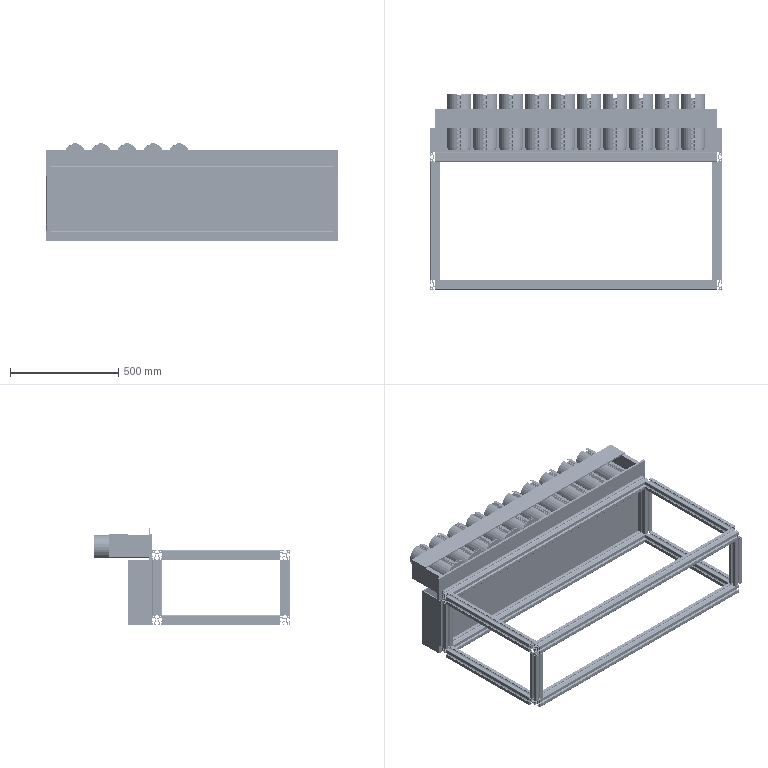Assembly | SolidWorks | mm | 438 component files | 477 solids | 23460 faces | box 1345 x 901.5 x 452.95 mm | volume 26250430 mm3 | cylinder 12408 | plane 6340 | torus 3280 | spline 860 | cone 572 | commonest cylinder face diameters 1 x1650 2.5 x1640 2 x1246 95.6 x1230 98.4 x1230 10 x976 6 x844 3.2 x820
Bill of materials:
Cover | 1 |  | Long, narrow, thin-walled rectangular trough or tray. A tall long wall runs the full length, with a closed end wall at each end and a bottom panel. The top and the long front side look open.
FeedingMechanism | 1 |  | Multi-body geometry: an open rectangular box frame made of slotted profile bars, with a long rectangular housing along one top edge that holds a row of evenly spaced parallel cylinders. A flat panel runs along one long side of the frame under the housing.
PusherTray | 2 |  | Long angle profile with an L-shaped cross-section: a tall thin vertical leg and a short horizontal foot, joined by a rounded inside and outside corner. The top of the tall leg narrows over a short taper.
5 | 4 |  | Socket-head-style fastener shape: a cylindrical head with a hexagonal recess and chamfered edges, on top of a shorter, smaller-diameter plain cylindrical shank with a chamfered tip.
6 | 4 |  | Elongated rectangular-section bar with rounded edges and a smaller cylindrical stub at one end. A thin strip and a small pin- or nut-like feature run along one side. The end view shows a rounded rectangular outline with a narrower raised tab carrying a chamfered cylindrical boss with a slot.
TR-20x75-SBaffle | 4 |  | Solid rectangular block with four through-holes on one face, in a row: a small hole near each end and two larger holes further in. One of the larger holes looks stepped (counterbored or shouldered).
TR-20x75-SCylinderBody | 4 |  | Rectangular body with lengthwise grooves on its long faces and two T-shaped undercut slots in one end profile. Two counterbored round openings and a hex-shaped fitting stick out of the top end. Small holes are spread over the side faces.
TR-20x75-SCylinderRod | 4 |  | Long, slender, solid cylindrical pin with a wider grooved collar at one end and a small notch or flat near the opposite tip. Seen end-on, the collar is circular, with a central section showing two parallel flats.
TR-20x75-SGuideRod | 4 |  | Long, slender tube-like pin, similar in shape to a grooved-collar pin. It has a central bore visible at the tip and a cone-bottomed bore seen from the end. The collar section shows a hexagon-like faceted outline.
WuliangyeBottleCap-1 | 410 |  | Thin flat plate with a mostly circular outline, a small rounded lobe at the top joined by concave fillets, and a straight-sided rectangular tab at the bottom. There are small holes near the tab corners.
Mates:
1. width | PusherTray-1 face at (575, 622.5, 22.5) dir (1, 0, 0) | PusherTray-1 face at (25, 628.5, 22.5) dir (-1, 0, 0) | FeedingMechanism-1 face at (452, 627.5, -157.5) dir (1, 0, 0) | FeedingMechanism-1 face at (148, 627.5, -157.5) dir (-1, 0, 0)
2. width | PusherTray-2 face at (-575, 628.5, 66.449) dir (-1, 0, 0) | PusherTray-2 face at (-25, 622.5, 66.449) dir (1, 0, 0) | FeedingMechanism-1 face at (-452, 627.5, -157.5) dir (-1, 0, 0) | FeedingMechanism-1 face at (-148, 627.5, -157.5) dir (1, 0, 0)
3. coincident | FeedingMechanism-1 face at (0, 622.5, 0) dir (0, 1, 0) | WuliangyeBottleCap-1-1 face at (517.1, 622.5, 143.39) dir (0, -1, 0)
4. concentric | FeedingMechanism-1 face at (540, 879, 187.5) dir (0, -1, 0) r 50 | WuliangyeBottleCap-1-1 face at (540, 622.5, 187.5) dir (0, 1, 0) r 49.2
5. parallel | FeedingMechanism-1 face at (0, 0, 247.479) dir (0, 0, 1) | WuliangyeBottleCap-1-387 face at (517.6, 856.5, 136.695) dir (0, 0, -1)
6. coincident | FeedingMechanism-1 face at (0, 627.5, 0) dir (0, 1, 0) | TR-20x75-S-GN-1 (0)1-1/TR-20x75-SCylinderBody-1 face at (-187.5, 627.5, -7.5) dir (0, -1, 0)
7. coincident | FeedingMechanism-1 edge at (-148, 622.5, -157.5) dir (-1, 0, 0) | TR-20x75-S-GN-1 (0)1-1/TR-20x75-SCylinderBody-1 face at (-180, 627.5, -157.5) dir (0, 0, -1)
8. coincident | FeedingMechanism-1 face at (-148, 627.5, -157.5) dir (1, 0, 0) | TR-20x75-S-GN-1 (0)1-1/TR-20x75-SCylinderBody-1 face at (-148, 628.2, -7.5) dir (1, 0, 0)
9. coincident | PusherTray-2 face at (-575, 628, 60.449) dir (0, 0, -1) | TR-20x75-S-GN-1 (0)1-1/TR-20x75-SBaffle-1 face at (-180, 628.5, 60.449) dir (0, 0, 1)
10. coincident | FeedingMechanism-1 face at (0, 627.5, 0) dir (0, 1, 0) | TR-20x75-S-GN-1 (0)1-2/TR-20x75-SCylinderBody-1 face at (-427.5, 627.5, -7.5) dir (0, -1, 0)
11. coincident | FeedingMechanism-1 face at (-388, 627.5, -157.5) dir (1, 0, 0) | TR-20x75-S-GN-1 (0)1-2/TR-20x75-SCylinderBody-1 face at (-388, 628.2, -7.5) dir (1, 0, 0)
12. coincident | FeedingMechanism-1 face at (-452, 627.5, -7.5) dir (0, 0, 1) | TR-20x75-S-GN-1 (0)1-2/TR-20x75-SCylinderBody-1 face at (-420, 627.5, -7.5) dir (0, 0, 1)
13. coincident | PusherTray-2 face at (-575, 651.5, 60.449) dir (0, 1, 0) | TR-20x75-S-GN-1 (0)1-2/TR-20x75-SBaffle-1 face at (-389.2, 651.5, 60.449) dir (0, 1, 0)
14. coincident | FeedingMechanism-1 face at (0, 627.5, 0) dir (0, 1, 0) | TR-20x75-S-GN-1 (0)-3/TR-20x75-SCylinderBody-1 face at (172.5, 627.5, -7.5) dir (0, -1, 0)
15. coincident | FeedingMechanism-1 face at (212, 627.5, -7.5) dir (0, 0, 1) | TR-20x75-S-GN-1 (0)-3/TR-20x75-SCylinderBody-1 face at (180, 627.5, -7.5) dir (0, 0, 1)
16. coincident | FeedingMechanism-1 face at (212, 627.5, -157.5) dir (1, 0, 0) | TR-20x75-S-GN-1 (0)-3/TR-20x75-SCylinderBody-1 face at (212, 628.2, -7.5) dir (1, 0, 0)
17. coincident | FeedingMechanism-1 face at (0, 627.5, 0) dir (0, 1, 0) | TR-20x75-S-GN-1 (0)-4/TR-20x75-SCylinderBody-1 face at (412.5, 627.5, -7.5) dir (0, -1, 0)
18. coincident | FeedingMechanism-1 face at (452, 627.5, -157.5) dir (1, 0, 0) | TR-20x75-S-GN-1 (0)-4/TR-20x75-SCylinderBody-1 face at (452, 628.2, -7.5) dir (1, 0, 0)
19. coincident | FeedingMechanism-1 face at (452, 627.5, -7.5) dir (0, 0, 1) | TR-20x75-S-GN-1 (0)-4/TR-20x75-SCylinderBody-1 face at (420, 627.5, -7.5) dir (0, 0, 1)
20. coincident | PusherTray-1 face at (25, 628, 16.5) dir (0, 0, -1) | TR-20x75-S-GN-1 (0)-4/TR-20x75-SBaffle-1 face at (420, 628.5, 16.5) dir (0, 0, 1)
21. coincident | PusherTray-1 face at (25, 651.5, 16.5) dir (0, 1, 0) | TR-20x75-S-GN-1 (0)-4/TR-20x75-SBaffle-1 face at (450.8, 651.5, 16.5) dir (0, 1, 0)
22. distance | WuliangyeBottleCap-1-401 face at (-82.9, 628.5, 143.39) dir (0, -1, 0) | FeedingMechanism-1 face at (0, 622.5, 0) dir (0, 1, 0)
23. concentric | FeedingMechanism-1 face at (-60, 879, 187.5) dir (0, -1, 0) r 50 | WuliangyeBottleCap-1-401 face at (-60, 628.5, 187.5) dir (0, 1, 0) r 49.2
24. parallel | FeedingMechanism-1 face at (-672.5, 622.5, 247.5) dir (0, 0, 1) | WuliangyeBottleCap-1-401 face at (-82.4, 628.5, 136.695) dir (0, 0, -1)
25. coincident | FeedingMechanism-1 face at (0, 622.5, 0) dir (0, 1, 0) | WuliangyeBottleCap-1-649 face at (-82.886, 622.5, 182.644) dir (0, -1, 0)
26. coincident | PusherTray-2 face at (-575, 628, 175.949) dir (0, 0, 1) | WuliangyeBottleCap-1-649 face at (-82.386, 622.5, 175.949) dir (0, 0, -1)
27. coincident | FeedingMechanism-1 face at (0, 622.5, 0) dir (0, 1, 0) | Cover-1 face at (0, 622.5, -22.5) dir (0, -1, 0)
28. coincident | FeedingMechanism-1 face at (672.5, 622.5, 247.5) dir (1, 0, 0) | Cover-1 face at (672.5, 722.5, 127.5) dir (1, 0, 0)
29. coincident | FeedingMechanism-1 face at (-672.5, 622.5, -172.5) dir (0, 0, -1) | Cover-1 face at (-672.5, 722.5, -172.5) dir (0, 0, -1)
30. distance | TR-20x75-SCylinderBody-1 face at (25.682, -34.061, -44.47) dir (-1, 0, 0) | TR-20x75-SBaffle-1 face at (-42.267, -34.061, -43.47) dir (-1, 0, 0)
31. concentric | TR-20x75-SBaffle-1 face at (-39.267, -48.061, -31.97) dir (1, 0, 0) r 5.5 | 5-1 face at (-31.974, -48.061, -31.97) dir (1, 0, 0) r 3
32. coincident | TR-20x75-SBaffle-1 face at (-36.267, -48.061, -27.62) dir (-1, 0, 0) | 5-1 face at (-36.267, -48.061, -28.17) dir (1, 0, 0)
33. coincident | TR-20x75-SCylinderBody-1 face at (25.682, -9.961, -24.77) dir (0, 0, 1) | 6-1 face at (27.682, -6.261, -24.77) dir (0, 0, -1)
34. coincident | TR-20x75-SCylinderBody-1 face at (25.682, -5.761, -24.37) dir (0, -1, 0) | 6-1 face at (27.682, -5.761, -21.07) dir (0, 1, 0)
35. distance | TR-20x75-SCylinderBody-1 face at (25.682, -34.061, -44.47) dir (-1, 0, 0) | 6-1 face at (27.682, -7.961, -24.77) dir (-1, 0, 0)
36. concentric | TR-20x75-SCylinderBody-1 face at (49.682, -48.061, -31.97) dir (1, 0, 0) r 5 | TR-20x75-SGuideRod-2 face at (39.983, -48.061, -31.97) dir (1, 0, 0) r 5
37. coincident | TR-20x75-SBaffle-1 face at (-30.267, -34.061, -43.47) dir (1, 0, 0) | TR-20x75-SGuideRod-2 face at (-30.267, -48.957, -29.906) dir (-1, 0, 0)
38. coincident | TR-20x75-SBaffle-1 face at (-42.267, -34.061, -43.47) dir (-1, 0, 0) | TR-20x75-SCylinderRod-1 face at (-42.267, -20.061, -29.72) dir (-1, 0, 0)
39. concentric | 5-1 face at (-31.974, -48.061, -31.97) dir (1, 0, 0) r 3 | TR-20x75-SGuideRod-2 face at (39.983, -48.061, -31.97) dir (1, 0, 0) r 5
40. concentric | TR-20x75-SBaffle-1 face at (-42.267, -20.061, -31.97) dir (1, 0, 0) r 785.398 | TR-20x75-SCylinderRod-1 face at (33.983, -20.061, -31.97) dir (1, 0, 0) r 5
41. concentric | TR-20x75-SCylinderBody-1 face at (49.682, -20.061, -31.97) dir (1, 0, 0) r 5 | TR-20x75-SCylinderRod-1 face at (33.983, -20.061, -31.97) dir (1, 0, 0) r 5
42. distance | TR-20x75-SCylinderBody-1 face at (25.682, -34.061, -44.47) dir (-1, 0, 0) | TR-20x75-SBaffle-1 face at (1.682, -34.061, -43.47) dir (-1, 0, 0)
43. concentric | TR-20x75-SBaffle-1 face at (4.682, -48.061, -31.97) dir (1, 0, 0) r 5.5 | 5-1 face at (11.975, -48.061, -31.97) dir (1, 0, 0) r 3
44. coincident | TR-20x75-SBaffle-1 face at (7.682, -48.061, -27.62) dir (-1, 0, 0) | 5-1 face at (7.682, -48.061, -28.17) dir (1, 0, 0)
45. coincident | TR-20x75-SCylinderBody-1 face at (25.682, -9.961, -24.77) dir (0, 0, 1) | 6-1 face at (27.682, -6.261, -24.77) dir (0, 0, -1)
46. coincident | TR-20x75-SCylinderBody-1 face at (25.682, -5.761, -24.37) dir (0, -1, 0) | 6-1 face at (27.682, -5.761, -21.07) dir (0, 1, 0)
47. distance | TR-20x75-SCylinderBody-1 face at (25.682, -34.061, -44.47) dir (-1, 0, 0) | 6-1 face at (27.682, -7.961, -24.77) dir (-1, 0, 0)
48. concentric | TR-20x75-SCylinderBody-1 face at (49.682, -48.061, -31.97) dir (1, 0, 0) r 5 | TR-20x75-SGuideRod-2 face at (83.932, -48.061, -31.97) dir (1, 0, 0) r 5
49. coincident | TR-20x75-SBaffle-1 face at (13.682, -34.061, -43.47) dir (1, 0, 0) | TR-20x75-SGuideRod-2 face at (13.682, -48.957, -29.906) dir (-1, 0, 0)
50. coincident | TR-20x75-SBaffle-1 face at (1.682, -34.061, -43.47) dir (-1, 0, 0) | TR-20x75-SCylinderRod-1 face at (1.682, -20.061, -29.72) dir (-1, 0, 0)
51. concentric | 5-1 face at (11.975, -48.061, -31.97) dir (1, 0, 0) r 3 | TR-20x75-SGuideRod-2 face at (83.932, -48.061, -31.97) dir (1, 0, 0) r 5
52. concentric | TR-20x75-SBaffle-1 face at (1.682, -20.061, -31.97) dir (1, 0, 0) r 785.398 | TR-20x75-SCylinderRod-1 face at (77.932, -20.061, -31.97) dir (1, 0, 0) r 5
53. concentric | TR-20x75-SCylinderBody-1 face at (49.682, -20.061, -31.97) dir (1, 0, 0) r 5 | TR-20x75-SCylinderRod-1 face at (77.932, -20.061, -31.97) dir (1, 0, 0) r 5